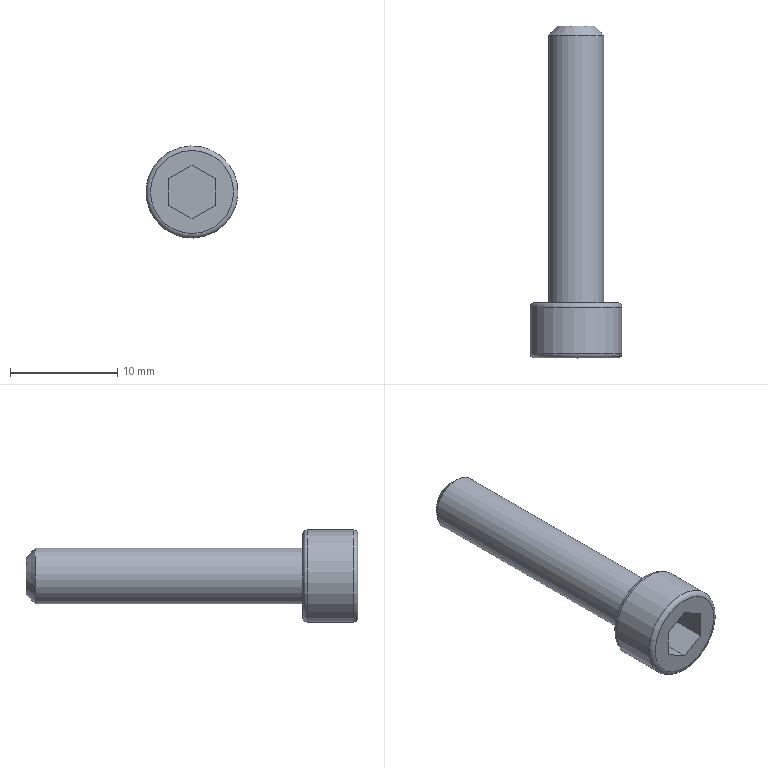Component | NX | M6X30_HEX_SCREW_3 | 1 solid | 15 faces | box 8.6 x 30.96 x 8.6 mm | volume 763 mm3 | plane 10 | cylinder 2 | torus 2 | cone 1 | commonest cylinder face diameters 5.16 x1 8.6 x1
STEP:
#1=CARTESIAN_POINT('',(0.,0.,0.));
#2=DIRECTION('',(0.,0.,1.));
#3=DIRECTION('',(1.,0.,0.));
#4=AXIS2_PLACEMENT_3D('',#1,#2,#3);
#5=CARTESIAN_POINT('',(-9.982,-499.433,-60.987));
#6=VERTEX_POINT('',#5);
#7=CARTESIAN_POINT('',(-11.917,-499.433,-57.635));
#8=DIRECTION('',(0.,-1.,0.));
#9=DIRECTION('',(0.5,0.,-0.866));
#10=AXIS2_PLACEMENT_3D('',#7,#8,#9);
#11=CIRCLE('',#10,3.87);
#12=CARTESIAN_POINT('',(-15.641,-499.433,-59.785));
#13=DIRECTION('',(0.,1.,0.));
#14=DIRECTION('',(0.5,0.,-0.866));
#15=AXIS2_PLACEMENT_3D('',#12,#13,#14);
#16=PLANE('',#15);
#17=CARTESIAN_POINT('',(3.87,-4.3));
#18=CARTESIAN_POINT('',(3.87,-11.003));
#19=CARTESIAN_POINT('',(-1.935,-7.652));
#20=CARTESIAN_POINT('',(-7.74,-4.3));
#21=CARTESIAN_POINT('',(-1.935,-0.9485));
#22=CARTESIAN_POINT('',(3.87,2.403));
#23=CARTESIAN_POINT('',(3.87,-4.3));
#24=(BOUNDED_CURVE()B_SPLINE_CURVE(2,(#17,#18,#19,#20,#21,#22,#23),.UNSPECIFIED.,.T.,.F.)B_SPLINE_CURVE_WITH_KNOTS((1,2,2,2,2,1),(-2.094,0.,2.094,4.189,6.283,8.378),.UNSPECIFIED.)CURVE()GEOMETRIC_REPRESENTATION_ITEM()RATIONAL_B_SPLINE_CURVE((1.,0.5,1.,0.5,1.,0.5,1.))REPRESENTATION_ITEM(''));
#25=(GEOMETRIC_REPRESENTATION_CONTEXT(2)PARAMETRIC_REPRESENTATION_CONTEXT()REPRESENTATION_CONTEXT('',''));
#26=DEFINITIONAL_REPRESENTATION('',(#24),#25);
#27=PCURVE('',#16,#26);
#28=CARTESIAN_POINT('',(-11.917,-499.003,-57.635));
#29=DIRECTION('',(0.,1.,0.));
#30=DIRECTION('',(0.5,0.,-0.866));
#31=AXIS2_PLACEMENT_3D('',#28,#29,#30);
#32=TOROIDAL_SURFACE('',#31,3.87,0.43);
#33=CARTESIAN_POINT('',(6.283,4.712));
#34=DIRECTION('',(-1.,0.));
#35=VECTOR('',#34,1.);
#36=LINE('',#33,#35);
#37=(GEOMETRIC_REPRESENTATION_CONTEXT(2)PARAMETRIC_REPRESENTATION_CONTEXT()REPRESENTATION_CONTEXT('',''));
#38=DEFINITIONAL_REPRESENTATION('',(#36),#37);
#39=PCURVE('',#32,#38);
#40=SURFACE_CURVE('',#11,(#27,#39),.PCURVE_S1.);
#41=EDGE_CURVE('',#6,#6,#40,.T.);
#42=ORIENTED_EDGE('',*,*,#41,.T.);
#43=EDGE_LOOP('',(#42));
#44=FACE_BOUND('',#43,.T.);
#45=CARTESIAN_POINT('',(-11.917,-499.433,-60.118));
#46=VERTEX_POINT('',#45);
#47=CARTESIAN_POINT('',(-9.767,-499.433,-58.877));
#48=VERTEX_POINT('',#47);
#49=CARTESIAN_POINT('',(-12.132,-499.433,-60.242));
#50=DIRECTION('',(0.866,0.,0.5));
#51=VECTOR('',#50,1.);
#52=LINE('',#49,#51);
#53=CARTESIAN_POINT('',(2.15,-2.81));
#54=DIRECTION('',(0.,-1.));
#55=VECTOR('',#54,1.);
#56=LINE('',#53,#55);
#57=(GEOMETRIC_REPRESENTATION_CONTEXT(2)PARAMETRIC_REPRESENTATION_CONTEXT()REPRESENTATION_CONTEXT('',''));
#58=DEFINITIONAL_REPRESENTATION('',(#56),#57);
#59=PCURVE('',#16,#58);
#60=CARTESIAN_POINT('',(-12.132,-495.133,-60.242));
#61=DIRECTION('',(0.5,0.,-0.866));
#62=DIRECTION('',(0.,-1.,0.));
#63=AXIS2_PLACEMENT_3D('',#60,#61,#62);
#64=PLANE('',#63);
#65=CARTESIAN_POINT('',(4.3,0.));
#66=DIRECTION('',(0.,-1.));
#67=VECTOR('',#66,1.);
#68=LINE('',#65,#67);
#69=(GEOMETRIC_REPRESENTATION_CONTEXT(2)PARAMETRIC_REPRESENTATION_CONTEXT()REPRESENTATION_CONTEXT('',''));
#70=DEFINITIONAL_REPRESENTATION('',(#68),#69);
#71=PCURVE('',#64,#70);
#72=SURFACE_CURVE('',#52,(#59,#71),.PCURVE_S1.);
#73=EDGE_CURVE('',#46,#48,#72,.T.);
#74=ORIENTED_EDGE('',*,*,#73,.F.);
#75=CARTESIAN_POINT('',(-14.067,-499.433,-58.877));
#76=VERTEX_POINT('',#75);
#77=CARTESIAN_POINT('',(-14.282,-499.433,-58.752));
#78=DIRECTION('',(0.866,0.,-0.5));
#79=VECTOR('',#78,1.);
#80=LINE('',#77,#79);
#81=CARTESIAN_POINT('',(-0.215,-1.693));
#82=DIRECTION('',(0.866,-0.5));
#83=VECTOR('',#82,1.);
#84=LINE('',#81,#83);
#85=(GEOMETRIC_REPRESENTATION_CONTEXT(2)PARAMETRIC_REPRESENTATION_CONTEXT()REPRESENTATION_CONTEXT('',''));
#86=DEFINITIONAL_REPRESENTATION('',(#84),#85);
#87=PCURVE('',#16,#86);
#88=CARTESIAN_POINT('',(-14.282,-495.133,-58.752));
#89=DIRECTION('',(-0.5,0.,-0.866));
#90=DIRECTION('',(0.866,0.,-0.5));
#91=AXIS2_PLACEMENT_3D('',#88,#89,#90);
#92=PLANE('',#91);
#93=CARTESIAN_POINT('',(0.,4.3));
#94=DIRECTION('',(1.,0.));
#95=VECTOR('',#94,1.);
#96=LINE('',#93,#95);
#97=(GEOMETRIC_REPRESENTATION_CONTEXT(2)PARAMETRIC_REPRESENTATION_CONTEXT()REPRESENTATION_CONTEXT('',''));
#98=DEFINITIONAL_REPRESENTATION('',(#96),#97);
#99=PCURVE('',#92,#98);
#100=SURFACE_CURVE('',#80,(#87,#99),.PCURVE_S1.);
#101=EDGE_CURVE('',#76,#46,#100,.T.);
#102=ORIENTED_EDGE('',*,*,#101,.F.);
#103=CARTESIAN_POINT('',(-14.067,-499.433,-56.394));
#104=VERTEX_POINT('',#103);
#105=CARTESIAN_POINT('',(-14.067,-499.433,-56.146));
#106=DIRECTION('',(-0.,0.,-1.));
#107=VECTOR('',#106,1.);
#108=LINE('',#105,#107);
#109=CARTESIAN_POINT('',(-2.365,-3.183));
#110=DIRECTION('',(0.866,0.5));
#111=VECTOR('',#110,1.);
#112=LINE('',#109,#111);
#113=(GEOMETRIC_REPRESENTATION_CONTEXT(2)PARAMETRIC_REPRESENTATION_CONTEXT()REPRESENTATION_CONTEXT('',''));
#114=DEFINITIONAL_REPRESENTATION('',(#112),#113);
#115=PCURVE('',#16,#114);
#116=CARTESIAN_POINT('',(-14.067,-495.133,-56.146));
#117=DIRECTION('',(-1.,0.,0.));
#118=DIRECTION('',(-0.,0.,-1.));
#119=AXIS2_PLACEMENT_3D('',#116,#117,#118);
#120=PLANE('',#119);
#121=CARTESIAN_POINT('',(0.,4.3));
#122=DIRECTION('',(1.,0.));
#123=VECTOR('',#122,1.);
#124=LINE('',#121,#123);
#125=(GEOMETRIC_REPRESENTATION_CONTEXT(2)PARAMETRIC_REPRESENTATION_CONTEXT()REPRESENTATION_CONTEXT('',''));
#126=DEFINITIONAL_REPRESENTATION('',(#124),#125);
#127=PCURVE('',#120,#126);
#128=SURFACE_CURVE('',#108,(#115,#127),.PCURVE_S1.);
#129=EDGE_CURVE('',#104,#76,#128,.T.);
#130=ORIENTED_EDGE('',*,*,#129,.F.);
#131=CARTESIAN_POINT('',(-11.917,-499.433,-55.153));
#132=VERTEX_POINT('',#131);
#133=CARTESIAN_POINT('',(-11.702,-499.433,-55.029));
#134=DIRECTION('',(-0.866,0.,-0.5));
#135=VECTOR('',#134,1.);
#136=LINE('',#133,#135);
#137=CARTESIAN_POINT('',(-2.15,-5.79));
#138=DIRECTION('',(0.,1.));
#139=VECTOR('',#138,1.);
#140=LINE('',#137,#139);
#141=(GEOMETRIC_REPRESENTATION_CONTEXT(2)PARAMETRIC_REPRESENTATION_CONTEXT()REPRESENTATION_CONTEXT('',''));
#142=DEFINITIONAL_REPRESENTATION('',(#140),#141);
#143=PCURVE('',#16,#142);
#144=CARTESIAN_POINT('',(-11.702,-495.133,-55.029));
#145=DIRECTION('',(-0.5,0.,0.866));
#146=DIRECTION('',(0.,1.,0.));
#147=AXIS2_PLACEMENT_3D('',#144,#145,#146);
#148=PLANE('',#147);
#149=CARTESIAN_POINT('',(-4.3,0.));
#150=DIRECTION('',(0.,1.));
#151=VECTOR('',#150,1.);
#152=LINE('',#149,#151);
#153=(GEOMETRIC_REPRESENTATION_CONTEXT(2)PARAMETRIC_REPRESENTATION_CONTEXT()REPRESENTATION_CONTEXT('',''));
#154=DEFINITIONAL_REPRESENTATION('',(#152),#153);
#155=PCURVE('',#148,#154);
#156=SURFACE_CURVE('',#136,(#143,#155),.PCURVE_S1.);
#157=EDGE_CURVE('',#132,#104,#156,.T.);
#158=ORIENTED_EDGE('',*,*,#157,.F.);
#159=CARTESIAN_POINT('',(-9.767,-499.433,-56.394));
#160=VERTEX_POINT('',#159);
#161=CARTESIAN_POINT('',(-9.552,-499.433,-56.518));
#162=DIRECTION('',(-0.866,0.,0.5));
#163=VECTOR('',#162,1.);
#164=LINE('',#161,#163);
#165=CARTESIAN_POINT('',(0.215,-6.907));
#166=DIRECTION('',(-0.866,0.5));
#167=VECTOR('',#166,1.);
#168=LINE('',#165,#167);
#169=(GEOMETRIC_REPRESENTATION_CONTEXT(2)PARAMETRIC_REPRESENTATION_CONTEXT()REPRESENTATION_CONTEXT('',''));
#170=DEFINITIONAL_REPRESENTATION('',(#168),#169);
#171=PCURVE('',#16,#170);
#172=CARTESIAN_POINT('',(-9.552,-495.133,-56.518));
#173=DIRECTION('',(0.5,0.,0.866));
#174=DIRECTION('',(-0.866,0.,0.5));
#175=AXIS2_PLACEMENT_3D('',#172,#173,#174);
#176=PLANE('',#175);
#177=CARTESIAN_POINT('',(0.,4.3));
#178=DIRECTION('',(1.,0.));
#179=VECTOR('',#178,1.);
#180=LINE('',#177,#179);
#181=(GEOMETRIC_REPRESENTATION_CONTEXT(2)PARAMETRIC_REPRESENTATION_CONTEXT()REPRESENTATION_CONTEXT('',''));
#182=DEFINITIONAL_REPRESENTATION('',(#180),#181);
#183=PCURVE('',#176,#182);
#184=SURFACE_CURVE('',#164,(#171,#183),.PCURVE_S1.);
#185=EDGE_CURVE('',#160,#132,#184,.T.);
#186=ORIENTED_EDGE('',*,*,#185,.F.);
#187=CARTESIAN_POINT('',(-9.767,-499.433,-59.125));
#188=DIRECTION('',(0.,0.,1.));
#189=VECTOR('',#188,1.);
#190=LINE('',#187,#189);
#191=CARTESIAN_POINT('',(2.365,-5.417));
#192=DIRECTION('',(-0.866,-0.5));
#193=VECTOR('',#192,1.);
#194=LINE('',#191,#193);
#195=(GEOMETRIC_REPRESENTATION_CONTEXT(2)PARAMETRIC_REPRESENTATION_CONTEXT()REPRESENTATION_CONTEXT('',''));
#196=DEFINITIONAL_REPRESENTATION('',(#194),#195);
#197=PCURVE('',#16,#196);
#198=CARTESIAN_POINT('',(-9.767,-495.133,-59.125));
#199=DIRECTION('',(1.,0.,-0.));
#200=DIRECTION('',(0.,0.,1.));
#201=AXIS2_PLACEMENT_3D('',#198,#199,#200);
#202=PLANE('',#201);
#203=CARTESIAN_POINT('',(0.,4.3));
#204=DIRECTION('',(1.,0.));
#205=VECTOR('',#204,1.);
#206=LINE('',#203,#205);
#207=(GEOMETRIC_REPRESENTATION_CONTEXT(2)PARAMETRIC_REPRESENTATION_CONTEXT()REPRESENTATION_CONTEXT('',''));
#208=DEFINITIONAL_REPRESENTATION('',(#206),#207);
#209=PCURVE('',#202,#208);
#210=SURFACE_CURVE('',#190,(#197,#209),.PCURVE_S1.);
#211=EDGE_CURVE('',#48,#160,#210,.T.);
#212=ORIENTED_EDGE('',*,*,#211,.F.);
#213=EDGE_LOOP('',(#74,#102,#130,#158,#186,#212));
#214=FACE_BOUND('',#213,.T.);
#215=ADVANCED_FACE('',(#44,#214),#16,.F.);
#216=CARTESIAN_POINT('',(-12.777,-468.473,-56.146));
#217=VERTEX_POINT('',#216);
#218=CARTESIAN_POINT('',(-11.917,-468.473,-57.635));
#219=DIRECTION('',(0.,1.,0.));
#220=DIRECTION('',(-0.5,0.,0.866));
#221=AXIS2_PLACEMENT_3D('',#218,#219,#220);
#222=CIRCLE('',#221,1.72);
#223=CARTESIAN_POINT('',(-11.917,-468.473,-57.635));
#224=DIRECTION('',(0.,-1.,0.));
#225=DIRECTION('',(-0.5,0.,0.866));
#226=AXIS2_PLACEMENT_3D('',#223,#224,#225);
#227=PLANE('',#226);
#228=CARTESIAN_POINT('',(1.72,-0.));
#229=CARTESIAN_POINT('',(1.72,-2.979));
#230=CARTESIAN_POINT('',(-0.86,-1.49));
#231=CARTESIAN_POINT('',(-3.44,0.));
#232=CARTESIAN_POINT('',(-0.86,1.49));
#233=CARTESIAN_POINT('',(1.72,2.979));
#234=CARTESIAN_POINT('',(1.72,-0.));
#235=(BOUNDED_CURVE()B_SPLINE_CURVE(2,(#228,#229,#230,#231,#232,#233,#234),.UNSPECIFIED.,.T.,.F.)B_SPLINE_CURVE_WITH_KNOTS((1,2,2,2,2,1),(-2.094,0.,2.094,4.189,6.283,8.378),.UNSPECIFIED.)CURVE()GEOMETRIC_REPRESENTATION_ITEM()RATIONAL_B_SPLINE_CURVE((1.,0.5,1.,0.5,1.,0.5,1.))REPRESENTATION_ITEM(''));
#236=(GEOMETRIC_REPRESENTATION_CONTEXT(2)PARAMETRIC_REPRESENTATION_CONTEXT()REPRESENTATION_CONTEXT('',''));
#237=DEFINITIONAL_REPRESENTATION('',(#235),#236);
#238=PCURVE('',#227,#237);
#239=CARTESIAN_POINT('',(-11.917,-469.333,-57.635));
#240=DIRECTION('',(0.,-1.,0.));
#241=DIRECTION('',(-0.5,0.,0.866));
#242=AXIS2_PLACEMENT_3D('',#239,#240,#241);
#243=CONICAL_SURFACE('',#242,2.58,0.7854);
#244=CARTESIAN_POINT('',(6.283,-0.86));
#245=DIRECTION('',(-1.,0.));
#246=VECTOR('',#245,1.);
#247=LINE('',#244,#246);
#248=(GEOMETRIC_REPRESENTATION_CONTEXT(2)PARAMETRIC_REPRESENTATION_CONTEXT()REPRESENTATION_CONTEXT('',''));
#249=DEFINITIONAL_REPRESENTATION('',(#247),#248);
#250=PCURVE('',#243,#249);
#251=SURFACE_CURVE('',#222,(#238,#250),.PCURVE_S1.);
#252=EDGE_CURVE('',#217,#217,#251,.T.);
#253=ORIENTED_EDGE('',*,*,#252,.T.);
#254=EDGE_LOOP('',(#253));
#255=FACE_BOUND('',#254,.T.);
#256=ADVANCED_FACE('',(#255),#227,.F.);
#257=CARTESIAN_POINT('',(-13.207,-469.333,-55.401));
#258=VERTEX_POINT('',#257);
#259=CARTESIAN_POINT('',(-11.917,-469.333,-57.635));
#260=DIRECTION('',(0.,-1.,0.));
#261=DIRECTION('',(-0.5,0.,0.866));
#262=AXIS2_PLACEMENT_3D('',#259,#260,#261);
#263=CIRCLE('',#262,2.58);
#264=CARTESIAN_POINT('',(-11.917,-468.473,-57.635));
#265=DIRECTION('',(0.,-1.,0.));
#266=DIRECTION('',(-0.5,0.,0.866));
#267=AXIS2_PLACEMENT_3D('',#264,#265,#266);
#268=CYLINDRICAL_SURFACE('',#267,2.58);
#269=CARTESIAN_POINT('',(0.,0.86));
#270=DIRECTION('',(1.,0.));
#271=VECTOR('',#270,1.);
#272=LINE('',#269,#271);
#273=(GEOMETRIC_REPRESENTATION_CONTEXT(2)PARAMETRIC_REPRESENTATION_CONTEXT()REPRESENTATION_CONTEXT('',''));
#274=DEFINITIONAL_REPRESENTATION('',(#272),#273);
#275=PCURVE('',#268,#274);
#276=CARTESIAN_POINT('',(0.,-0.));
#277=DIRECTION('',(1.,0.));
#278=VECTOR('',#277,1.);
#279=LINE('',#276,#278);
#280=(GEOMETRIC_REPRESENTATION_CONTEXT(2)PARAMETRIC_REPRESENTATION_CONTEXT()REPRESENTATION_CONTEXT('',''));
#281=DEFINITIONAL_REPRESENTATION('',(#279),#280);
#282=PCURVE('',#243,#281);
#283=SURFACE_CURVE('',#263,(#275,#282),.PCURVE_S1.);
#284=EDGE_CURVE('',#258,#258,#283,.T.);
#285=ORIENTED_EDGE('',*,*,#284,.T.);
#286=CARTESIAN_POINT('',(-13.207,-494.273,-55.401));
#287=VERTEX_POINT('',#286);
#288=CARTESIAN_POINT('',(-13.207,-469.333,-55.401));
#289=CARTESIAN_POINT('',(-13.207,-494.273,-55.401));
#290=B_SPLINE_CURVE_WITH_KNOTS('',1,(#288,#289),.UNSPECIFIED.,.F.,.F.,(2,2),(0.86,25.8),.PIECEWISE_BEZIER_KNOTS.);
#291=CARTESIAN_POINT('',(6.283,0.));
#292=DIRECTION('',(0.,1.));
#293=VECTOR('',#292,1.);
#294=LINE('',#291,#293);
#295=(GEOMETRIC_REPRESENTATION_CONTEXT(2)PARAMETRIC_REPRESENTATION_CONTEXT()REPRESENTATION_CONTEXT('',''));
#296=DEFINITIONAL_REPRESENTATION('',(#294),#295);
#297=PCURVE('',#268,#296);
#298=CARTESIAN_POINT('',(0.,0.));
#299=DIRECTION('',(0.,1.));
#300=VECTOR('',#299,1.);
#301=LINE('',#298,#300);
#302=(GEOMETRIC_REPRESENTATION_CONTEXT(2)PARAMETRIC_REPRESENTATION_CONTEXT()REPRESENTATION_CONTEXT('',''));
#303=DEFINITIONAL_REPRESENTATION('',(#301),#302);
#304=PCURVE('',#268,#303);
#305=SEAM_CURVE('',#290,(#297,#304),.PCURVE_S1.);
#306=EDGE_CURVE('',#258,#287,#305,.T.);
#307=ORIENTED_EDGE('',*,*,#306,.T.);
#308=CARTESIAN_POINT('',(-11.917,-494.273,-57.635));
#309=DIRECTION('',(0.,-1.,0.));
#310=DIRECTION('',(-0.5,0.,0.866));
#311=AXIS2_PLACEMENT_3D('',#308,#309,#310);
#312=CIRCLE('',#311,2.58);
#313=CARTESIAN_POINT('',(0.,25.8));
#314=DIRECTION('',(1.,0.));
#315=VECTOR('',#314,1.);
#316=LINE('',#313,#315);
#317=(GEOMETRIC_REPRESENTATION_CONTEXT(2)PARAMETRIC_REPRESENTATION_CONTEXT()REPRESENTATION_CONTEXT('',''));
#318=DEFINITIONAL_REPRESENTATION('',(#316),#317);
#319=PCURVE('',#268,#318);
#320=CARTESIAN_POINT('',(-14.151,-494.273,-58.925));
#321=DIRECTION('',(0.,-1.,0.));
#322=DIRECTION('',(-0.5,0.,0.866));
#323=AXIS2_PLACEMENT_3D('',#320,#321,#322);
#324=PLANE('',#323);
#325=CARTESIAN_POINT('',(-0.,-2.58));
#326=DIRECTION('',(1.,-0.));
#327=AXIS2_PLACEMENT_2D('',#325,#326);
#328=CIRCLE('',#327,2.58);
#329=(GEOMETRIC_REPRESENTATION_CONTEXT(2)PARAMETRIC_REPRESENTATION_CONTEXT()REPRESENTATION_CONTEXT('',''));
#330=DEFINITIONAL_REPRESENTATION('',(#328),#329);
#331=PCURVE('',#324,#330);
#332=SURFACE_CURVE('',#312,(#319,#331),.PCURVE_S1.);
#333=EDGE_CURVE('',#287,#287,#332,.T.);
#334=ORIENTED_EDGE('',*,*,#333,.F.);
#335=ORIENTED_EDGE('',*,*,#306,.F.);
#336=EDGE_LOOP('',(#285,#307,#334,#335));
#337=FACE_BOUND('',#336,.T.);
#338=ADVANCED_FACE('',(#337),#268,.T.);
#339=CARTESIAN_POINT('',(-13.852,-494.273,-54.284));
#340=VERTEX_POINT('',#339);
#341=CARTESIAN_POINT('',(-11.917,-494.273,-57.635));
#342=DIRECTION('',(0.,1.,0.));
#343=DIRECTION('',(-0.5,0.,0.866));
#344=AXIS2_PLACEMENT_3D('',#341,#342,#343);
#345=CIRCLE('',#344,3.87);
#346=CARTESIAN_POINT('',(3.87,-2.58));
#347=CARTESIAN_POINT('',(3.87,-9.283));
#348=CARTESIAN_POINT('',(-1.935,-5.932));
#349=CARTESIAN_POINT('',(-7.74,-2.58));
#350=CARTESIAN_POINT('',(-1.935,0.7715));
#351=CARTESIAN_POINT('',(3.87,4.123));
#352=CARTESIAN_POINT('',(3.87,-2.58));
#353=(BOUNDED_CURVE()B_SPLINE_CURVE(2,(#346,#347,#348,#349,#350,#351,#352),.UNSPECIFIED.,.T.,.F.)B_SPLINE_CURVE_WITH_KNOTS((1,2,2,2,2,1),(-2.094,0.,2.094,4.189,6.283,8.378),.UNSPECIFIED.)CURVE()GEOMETRIC_REPRESENTATION_ITEM()RATIONAL_B_SPLINE_CURVE((1.,0.5,1.,0.5,1.,0.5,1.))REPRESENTATION_ITEM(''));
#354=(GEOMETRIC_REPRESENTATION_CONTEXT(2)PARAMETRIC_REPRESENTATION_CONTEXT()REPRESENTATION_CONTEXT('',''));
#355=DEFINITIONAL_REPRESENTATION('',(#353),#354);
#356=PCURVE('',#324,#355);
#357=CARTESIAN_POINT('',(-11.917,-494.703,-57.635));
#358=DIRECTION('',(0.,-1.,0.));
#359=DIRECTION('',(-0.5,0.,0.866));
#360=AXIS2_PLACEMENT_3D('',#357,#358,#359);
#361=TOROIDAL_SURFACE('',#360,3.87,0.43);
#362=CARTESIAN_POINT('',(6.283,4.712));
#363=DIRECTION('',(-1.,0.));
#364=VECTOR('',#363,1.);
#365=LINE('',#362,#364);
#366=(GEOMETRIC_REPRESENTATION_CONTEXT(2)PARAMETRIC_REPRESENTATION_CONTEXT()REPRESENTATION_CONTEXT('',''));
#367=DEFINITIONAL_REPRESENTATION('',(#365),#366);
#368=PCURVE('',#361,#367);
#369=SURFACE_CURVE('',#345,(#356,#368),.PCURVE_S1.);
#370=EDGE_CURVE('',#340,#340,#369,.T.);
#371=ORIENTED_EDGE('',*,*,#370,.T.);
#372=EDGE_LOOP('',(#371));
#373=FACE_BOUND('',#372,.T.);
#374=ORIENTED_EDGE('',*,*,#333,.T.);
#375=EDGE_LOOP('',(#374));
#376=FACE_BOUND('',#375,.T.);
#377=ADVANCED_FACE('',(#373,#376),#324,.F.);
#378=CARTESIAN_POINT('',(-14.067,-494.703,-53.911));
#379=VERTEX_POINT('',#378);
#380=CARTESIAN_POINT('',(-11.917,-494.703,-57.635));
#381=DIRECTION('',(0.,-1.,0.));
#382=DIRECTION('',(-0.5,0.,0.866));
#383=AXIS2_PLACEMENT_3D('',#380,#381,#382);
#384=CIRCLE('',#383,4.3);
#385=CARTESIAN_POINT('',(-11.917,-468.473,-57.635));
#386=DIRECTION('',(0.,-1.,0.));
#387=DIRECTION('',(-0.5,0.,0.866));
#388=AXIS2_PLACEMENT_3D('',#385,#386,#387);
#389=CYLINDRICAL_SURFACE('',#388,4.3);
#390=CARTESIAN_POINT('',(0.,26.23));
#391=DIRECTION('',(1.,0.));
#392=VECTOR('',#391,1.);
#393=LINE('',#390,#392);
#394=(GEOMETRIC_REPRESENTATION_CONTEXT(2)PARAMETRIC_REPRESENTATION_CONTEXT()REPRESENTATION_CONTEXT('',''));
#395=DEFINITIONAL_REPRESENTATION('',(#393),#394);
#396=PCURVE('',#389,#395);
#397=CARTESIAN_POINT('',(0.,6.283));
#398=DIRECTION('',(1.,0.));
#399=VECTOR('',#398,1.);
#400=LINE('',#397,#399);
#401=(GEOMETRIC_REPRESENTATION_CONTEXT(2)PARAMETRIC_REPRESENTATION_CONTEXT()REPRESENTATION_CONTEXT('',''));
#402=DEFINITIONAL_REPRESENTATION('',(#400),#401);
#403=PCURVE('',#361,#402);
#404=SURFACE_CURVE('',#384,(#396,#403),.PCURVE_S1.);
#405=EDGE_CURVE('',#379,#379,#404,.T.);
#406=ORIENTED_EDGE('',*,*,#405,.T.);
#407=CARTESIAN_POINT('',(-14.067,-499.003,-53.911));
#408=VERTEX_POINT('',#407);
#409=CARTESIAN_POINT('',(-14.067,-494.703,-53.911));
#410=CARTESIAN_POINT('',(-14.067,-499.003,-53.911));
#411=B_SPLINE_CURVE_WITH_KNOTS('',1,(#409,#410),.UNSPECIFIED.,.F.,.F.,(2,2),(26.23,30.53),.PIECEWISE_BEZIER_KNOTS.);
#412=CARTESIAN_POINT('',(6.283,0.));
#413=DIRECTION('',(0.,1.));
#414=VECTOR('',#413,1.);
#415=LINE('',#412,#414);
#416=(GEOMETRIC_REPRESENTATION_CONTEXT(2)PARAMETRIC_REPRESENTATION_CONTEXT()REPRESENTATION_CONTEXT('',''));
#417=DEFINITIONAL_REPRESENTATION('',(#415),#416);
#418=PCURVE('',#389,#417);
#419=CARTESIAN_POINT('',(0.,0.));
#420=DIRECTION('',(0.,1.));
#421=VECTOR('',#420,1.);
#422=LINE('',#419,#421);
#423=(GEOMETRIC_REPRESENTATION_CONTEXT(2)PARAMETRIC_REPRESENTATION_CONTEXT()REPRESENTATION_CONTEXT('',''));
#424=DEFINITIONAL_REPRESENTATION('',(#422),#423);
#425=PCURVE('',#389,#424);
#426=SEAM_CURVE('',#411,(#418,#425),.PCURVE_S1.);
#427=EDGE_CURVE('',#379,#408,#426,.T.);
#428=ORIENTED_EDGE('',*,*,#427,.T.);
#429=CARTESIAN_POINT('',(-9.767,-499.003,-61.359));
#430=VERTEX_POINT('',#429);
#431=CARTESIAN_POINT('',(-11.917,-499.003,-57.635));
#432=DIRECTION('',(0.,1.,0.));
#433=DIRECTION('',(0.5,0.,-0.866));
#434=AXIS2_PLACEMENT_3D('',#431,#432,#433);
#435=CIRCLE('',#434,4.3);
#436=CARTESIAN_POINT('',(9.425,30.53));
#437=DIRECTION('',(-1.,0.));
#438=VECTOR('',#437,1.);
#439=LINE('',#436,#438);
#440=(GEOMETRIC_REPRESENTATION_CONTEXT(2)PARAMETRIC_REPRESENTATION_CONTEXT()REPRESENTATION_CONTEXT('',''));
#441=DEFINITIONAL_REPRESENTATION('',(#439),#440);
#442=PCURVE('',#389,#441);
#443=CARTESIAN_POINT('',(0.,6.283));
#444=DIRECTION('',(1.,0.));
#445=VECTOR('',#444,1.);
#446=LINE('',#443,#445);
#447=(GEOMETRIC_REPRESENTATION_CONTEXT(2)PARAMETRIC_REPRESENTATION_CONTEXT()REPRESENTATION_CONTEXT('',''));
#448=DEFINITIONAL_REPRESENTATION('',(#446),#447);
#449=PCURVE('',#32,#448);
#450=SURFACE_CURVE('',#435,(#442,#449),.PCURVE_S1.);
#451=EDGE_CURVE('',#408,#430,#450,.T.);
#452=ORIENTED_EDGE('',*,*,#451,.T.);
#453=CARTESIAN_POINT('',(-11.917,-499.003,-57.635));
#454=DIRECTION('',(0.,1.,0.));
#455=DIRECTION('',(0.5,0.,-0.866));
#456=AXIS2_PLACEMENT_3D('',#453,#454,#455);
#457=CIRCLE('',#456,4.3);
#458=CARTESIAN_POINT('',(3.142,30.53));
#459=DIRECTION('',(-1.,0.));
#460=VECTOR('',#459,1.);
#461=LINE('',#458,#460);
#462=(GEOMETRIC_REPRESENTATION_CONTEXT(2)PARAMETRIC_REPRESENTATION_CONTEXT()REPRESENTATION_CONTEXT('',''));
#463=DEFINITIONAL_REPRESENTATION('',(#461),#462);
#464=PCURVE('',#389,#463);
#465=CARTESIAN_POINT('',(0.,6.283));
#466=DIRECTION('',(1.,0.));
#467=VECTOR('',#466,1.);
#468=LINE('',#465,#467);
#469=(GEOMETRIC_REPRESENTATION_CONTEXT(2)PARAMETRIC_REPRESENTATION_CONTEXT()REPRESENTATION_CONTEXT('',''));
#470=DEFINITIONAL_REPRESENTATION('',(#468),#469);
#471=PCURVE('',#32,#470);
#472=SURFACE_CURVE('',#457,(#464,#471),.PCURVE_S1.);
#473=EDGE_CURVE('',#430,#408,#472,.T.);
#474=ORIENTED_EDGE('',*,*,#473,.T.);
#475=ORIENTED_EDGE('',*,*,#427,.F.);
#476=EDGE_LOOP('',(#406,#428,#452,#474,#475));
#477=FACE_BOUND('',#476,.T.);
#478=ADVANCED_FACE('',(#477),#389,.T.);
#479=ORIENTED_EDGE('',*,*,#73,.T.);
#480=CARTESIAN_POINT('',(-9.767,-495.133,-58.877));
#481=VERTEX_POINT('',#480);
#482=CARTESIAN_POINT('',(-9.767,-495.133,-58.877));
#483=DIRECTION('',(0.,1.,0.));
#484=VECTOR('',#483,1.);
#485=LINE('',#482,#484);
#486=CARTESIAN_POINT('',(0.,-2.731));
#487=DIRECTION('',(-1.,0.));
#488=VECTOR('',#487,1.);
#489=LINE('',#486,#488);
#490=(GEOMETRIC_REPRESENTATION_CONTEXT(2)PARAMETRIC_REPRESENTATION_CONTEXT()REPRESENTATION_CONTEXT('',''));
#491=DEFINITIONAL_REPRESENTATION('',(#489),#490);
#492=PCURVE('',#64,#491);
#493=CARTESIAN_POINT('',(0.2483,0.));
#494=DIRECTION('',(0.,-1.));
#495=VECTOR('',#494,1.);
#496=LINE('',#493,#495);
#497=(GEOMETRIC_REPRESENTATION_CONTEXT(2)PARAMETRIC_REPRESENTATION_CONTEXT()REPRESENTATION_CONTEXT('',''));
#498=DEFINITIONAL_REPRESENTATION('',(#496),#497);
#499=PCURVE('',#202,#498);
#500=SURFACE_CURVE('',#485,(#492,#499),.PCURVE_S1.);
#501=EDGE_CURVE('',#48,#481,#500,.T.);
#502=ORIENTED_EDGE('',*,*,#501,.T.);
#503=CARTESIAN_POINT('',(-11.917,-495.133,-60.118));
#504=VERTEX_POINT('',#503);
#505=CARTESIAN_POINT('',(-12.132,-495.133,-60.242));
#506=DIRECTION('',(-0.866,0.,-0.5));
#507=VECTOR('',#506,1.);
#508=LINE('',#505,#507);
#509=CARTESIAN_POINT('',(0.,0.));
#510=DIRECTION('',(0.,1.));
#511=VECTOR('',#510,1.);
#512=LINE('',#509,#511);
#513=(GEOMETRIC_REPRESENTATION_CONTEXT(2)PARAMETRIC_REPRESENTATION_CONTEXT()REPRESENTATION_CONTEXT('',''));
#514=DEFINITIONAL_REPRESENTATION('',(#512),#513);
#515=PCURVE('',#64,#514);
#516=CARTESIAN_POINT('',(-11.917,-495.133,-57.635));
#517=DIRECTION('',(0.,-1.,0.));
#518=DIRECTION('',(-0.5,0.,0.866));
#519=AXIS2_PLACEMENT_3D('',#516,#517,#518);
#520=PLANE('',#519);
#521=CARTESIAN_POINT('',(-2.15,1.49));
#522=DIRECTION('',(0.,1.));
#523=VECTOR('',#522,1.);
#524=LINE('',#521,#523);
#525=(GEOMETRIC_REPRESENTATION_CONTEXT(2)PARAMETRIC_REPRESENTATION_CONTEXT()REPRESENTATION_CONTEXT('',''));
#526=DEFINITIONAL_REPRESENTATION('',(#524),#525);
#527=PCURVE('',#520,#526);
#528=SURFACE_CURVE('',#508,(#515,#527),.PCURVE_S1.);
#529=EDGE_CURVE('',#481,#504,#528,.T.);
#530=ORIENTED_EDGE('',*,*,#529,.T.);
#531=CARTESIAN_POINT('',(-11.917,-495.133,-60.118));
#532=DIRECTION('',(0.,1.,0.));
#533=VECTOR('',#532,1.);
#534=LINE('',#531,#533);
#535=CARTESIAN_POINT('',(0.,-0.2483));
#536=DIRECTION('',(-1.,0.));
#537=VECTOR('',#536,1.);
#538=LINE('',#535,#537);
#539=(GEOMETRIC_REPRESENTATION_CONTEXT(2)PARAMETRIC_REPRESENTATION_CONTEXT()REPRESENTATION_CONTEXT('',''));
#540=DEFINITIONAL_REPRESENTATION('',(#538),#539);
#541=PCURVE('',#64,#540);
#542=CARTESIAN_POINT('',(2.731,0.));
#543=DIRECTION('',(0.,-1.));
#544=VECTOR('',#543,1.);
#545=LINE('',#542,#544);
#546=(GEOMETRIC_REPRESENTATION_CONTEXT(2)PARAMETRIC_REPRESENTATION_CONTEXT()REPRESENTATION_CONTEXT('',''));
#547=DEFINITIONAL_REPRESENTATION('',(#545),#546);
#548=PCURVE('',#92,#547);
#549=SURFACE_CURVE('',#534,(#541,#548),.PCURVE_S1.);
#550=EDGE_CURVE('',#46,#504,#549,.T.);
#551=ORIENTED_EDGE('',*,*,#550,.F.);
#552=EDGE_LOOP('',(#479,#502,#530,#551));
#553=FACE_BOUND('',#552,.T.);
#554=ADVANCED_FACE('',(#553),#64,.F.);
#555=ORIENTED_EDGE('',*,*,#211,.T.);
#556=CARTESIAN_POINT('',(-9.767,-495.133,-56.394));
#557=VERTEX_POINT('',#556);
#558=CARTESIAN_POINT('',(-9.767,-495.133,-56.394));
#559=DIRECTION('',(0.,1.,0.));
#560=VECTOR('',#559,1.);
#561=LINE('',#558,#560);
#562=CARTESIAN_POINT('',(2.731,0.));
#563=DIRECTION('',(0.,-1.));
#564=VECTOR('',#563,1.);
#565=LINE('',#562,#564);
#566=(GEOMETRIC_REPRESENTATION_CONTEXT(2)PARAMETRIC_REPRESENTATION_CONTEXT()REPRESENTATION_CONTEXT('',''));
#567=DEFINITIONAL_REPRESENTATION('',(#565),#566);
#568=PCURVE('',#202,#567);
#569=CARTESIAN_POINT('',(0.2483,0.));
#570=DIRECTION('',(0.,-1.));
#571=VECTOR('',#570,1.);
#572=LINE('',#569,#571);
#573=(GEOMETRIC_REPRESENTATION_CONTEXT(2)PARAMETRIC_REPRESENTATION_CONTEXT()REPRESENTATION_CONTEXT('',''));
#574=DEFINITIONAL_REPRESENTATION('',(#572),#573);
#575=PCURVE('',#176,#574);
#576=SURFACE_CURVE('',#561,(#568,#575),.PCURVE_S1.);
#577=EDGE_CURVE('',#160,#557,#576,.T.);
#578=ORIENTED_EDGE('',*,*,#577,.T.);
#579=CARTESIAN_POINT('',(-9.767,-495.133,-59.125));
#580=DIRECTION('',(-0.,0.,-1.));
#581=VECTOR('',#580,1.);
#582=LINE('',#579,#581);
#583=CARTESIAN_POINT('',(0.,0.));
#584=DIRECTION('',(-1.,0.));
#585=VECTOR('',#584,1.);
#586=LINE('',#583,#585);
#587=(GEOMETRIC_REPRESENTATION_CONTEXT(2)PARAMETRIC_REPRESENTATION_CONTEXT()REPRESENTATION_CONTEXT('',''));
#588=DEFINITIONAL_REPRESENTATION('',(#586),#587);
#589=PCURVE('',#202,#588);
#590=CARTESIAN_POINT('',(-2.365,-1.117));
#591=DIRECTION('',(-0.866,0.5));
#592=VECTOR('',#591,1.);
#593=LINE('',#590,#592);
#594=(GEOMETRIC_REPRESENTATION_CONTEXT(2)PARAMETRIC_REPRESENTATION_CONTEXT()REPRESENTATION_CONTEXT('',''));
#595=DEFINITIONAL_REPRESENTATION('',(#593),#594);
#596=PCURVE('',#520,#595);
#597=SURFACE_CURVE('',#582,(#589,#596),.PCURVE_S1.);
#598=EDGE_CURVE('',#557,#481,#597,.T.);
#599=ORIENTED_EDGE('',*,*,#598,.T.);
#600=ORIENTED_EDGE('',*,*,#501,.F.);
#601=EDGE_LOOP('',(#555,#578,#599,#600));
#602=FACE_BOUND('',#601,.T.);
#603=ADVANCED_FACE('',(#602),#202,.F.);
#604=ORIENTED_EDGE('',*,*,#185,.T.);
#605=CARTESIAN_POINT('',(-11.917,-495.133,-55.153));
#606=VERTEX_POINT('',#605);
#607=CARTESIAN_POINT('',(-11.917,-495.133,-55.153));
#608=DIRECTION('',(0.,1.,0.));
#609=VECTOR('',#608,1.);
#610=LINE('',#607,#609);
#611=CARTESIAN_POINT('',(2.731,0.));
#612=DIRECTION('',(0.,-1.));
#613=VECTOR('',#612,1.);
#614=LINE('',#611,#613);
#615=(GEOMETRIC_REPRESENTATION_CONTEXT(2)PARAMETRIC_REPRESENTATION_CONTEXT()REPRESENTATION_CONTEXT('',''));
#616=DEFINITIONAL_REPRESENTATION('',(#614),#615);
#617=PCURVE('',#176,#616);
#618=CARTESIAN_POINT('',(0.,0.2483));
#619=DIRECTION('',(1.,0.));
#620=VECTOR('',#619,1.);
#621=LINE('',#618,#620);
#622=(GEOMETRIC_REPRESENTATION_CONTEXT(2)PARAMETRIC_REPRESENTATION_CONTEXT()REPRESENTATION_CONTEXT('',''));
#623=DEFINITIONAL_REPRESENTATION('',(#621),#622);
#624=PCURVE('',#148,#623);
#625=SURFACE_CURVE('',#610,(#617,#624),.PCURVE_S1.);
#626=EDGE_CURVE('',#132,#606,#625,.T.);
#627=ORIENTED_EDGE('',*,*,#626,.T.);
#628=CARTESIAN_POINT('',(-9.552,-495.133,-56.518));
#629=DIRECTION('',(0.866,0.,-0.5));
#630=VECTOR('',#629,1.);
#631=LINE('',#628,#630);
#632=CARTESIAN_POINT('',(0.,0.));
#633=DIRECTION('',(-1.,0.));
#634=VECTOR('',#633,1.);
#635=LINE('',#632,#634);
#636=(GEOMETRIC_REPRESENTATION_CONTEXT(2)PARAMETRIC_REPRESENTATION_CONTEXT()REPRESENTATION_CONTEXT('',''));
#637=DEFINITIONAL_REPRESENTATION('',(#635),#636);
#638=PCURVE('',#176,#637);
#639=CARTESIAN_POINT('',(-0.215,-2.607));
#640=DIRECTION('',(-0.866,-0.5));
#641=VECTOR('',#640,1.);
#642=LINE('',#639,#641);
#643=(GEOMETRIC_REPRESENTATION_CONTEXT(2)PARAMETRIC_REPRESENTATION_CONTEXT()REPRESENTATION_CONTEXT('',''));
#644=DEFINITIONAL_REPRESENTATION('',(#642),#643);
#645=PCURVE('',#520,#644);
#646=SURFACE_CURVE('',#631,(#638,#645),.PCURVE_S1.);
#647=EDGE_CURVE('',#606,#557,#646,.T.);
#648=ORIENTED_EDGE('',*,*,#647,.T.);
#649=ORIENTED_EDGE('',*,*,#577,.F.);
#650=EDGE_LOOP('',(#604,#627,#648,#649));
#651=FACE_BOUND('',#650,.T.);
#652=ADVANCED_FACE('',(#651),#176,.F.);
#653=ORIENTED_EDGE('',*,*,#157,.T.);
#654=CARTESIAN_POINT('',(-14.067,-495.133,-56.394));
#655=VERTEX_POINT('',#654);
#656=CARTESIAN_POINT('',(-14.067,-495.133,-56.394));
#657=DIRECTION('',(0.,1.,0.));
#658=VECTOR('',#657,1.);
#659=LINE('',#656,#658);
#660=CARTESIAN_POINT('',(0.,2.731));
#661=DIRECTION('',(1.,0.));
#662=VECTOR('',#661,1.);
#663=LINE('',#660,#662);
#664=(GEOMETRIC_REPRESENTATION_CONTEXT(2)PARAMETRIC_REPRESENTATION_CONTEXT()REPRESENTATION_CONTEXT('',''));
#665=DEFINITIONAL_REPRESENTATION('',(#663),#664);
#666=PCURVE('',#148,#665);
#667=CARTESIAN_POINT('',(0.2483,0.));
#668=DIRECTION('',(0.,-1.));
#669=VECTOR('',#668,1.);
#670=LINE('',#667,#669);
#671=(GEOMETRIC_REPRESENTATION_CONTEXT(2)PARAMETRIC_REPRESENTATION_CONTEXT()REPRESENTATION_CONTEXT('',''));
#672=DEFINITIONAL_REPRESENTATION('',(#670),#671);
#673=PCURVE('',#120,#672);
#674=SURFACE_CURVE('',#659,(#666,#673),.PCURVE_S1.);
#675=EDGE_CURVE('',#104,#655,#674,.T.);
#676=ORIENTED_EDGE('',*,*,#675,.T.);
#677=CARTESIAN_POINT('',(-11.702,-495.133,-55.029));
#678=DIRECTION('',(0.866,0.,0.5));
#679=VECTOR('',#678,1.);
#680=LINE('',#677,#679);
#681=CARTESIAN_POINT('',(0.,0.));
#682=DIRECTION('',(0.,-1.));
#683=VECTOR('',#682,1.);
#684=LINE('',#681,#683);
#685=(GEOMETRIC_REPRESENTATION_CONTEXT(2)PARAMETRIC_REPRESENTATION_CONTEXT()REPRESENTATION_CONTEXT('',''));
#686=DEFINITIONAL_REPRESENTATION('',(#684),#685);
#687=PCURVE('',#148,#686);
#688=CARTESIAN_POINT('',(2.15,-1.49));
#689=DIRECTION('',(0.,-1.));
#690=VECTOR('',#689,1.);
#691=LINE('',#688,#690);
#692=(GEOMETRIC_REPRESENTATION_CONTEXT(2)PARAMETRIC_REPRESENTATION_CONTEXT()REPRESENTATION_CONTEXT('',''));
#693=DEFINITIONAL_REPRESENTATION('',(#691),#692);
#694=PCURVE('',#520,#693);
#695=SURFACE_CURVE('',#680,(#687,#694),.PCURVE_S1.);
#696=EDGE_CURVE('',#655,#606,#695,.T.);
#697=ORIENTED_EDGE('',*,*,#696,.T.);
#698=ORIENTED_EDGE('',*,*,#626,.F.);
#699=EDGE_LOOP('',(#653,#676,#697,#698));
#700=FACE_BOUND('',#699,.T.);
#701=ADVANCED_FACE('',(#700),#148,.F.);
#702=ORIENTED_EDGE('',*,*,#129,.T.);
#703=CARTESIAN_POINT('',(-14.067,-495.133,-58.877));
#704=VERTEX_POINT('',#703);
#705=CARTESIAN_POINT('',(-14.067,-495.133,-58.877));
#706=DIRECTION('',(0.,1.,0.));
#707=VECTOR('',#706,1.);
#708=LINE('',#705,#707);
#709=CARTESIAN_POINT('',(2.731,0.));
#710=DIRECTION('',(0.,-1.));
#711=VECTOR('',#710,1.);
#712=LINE('',#709,#711);
#713=(GEOMETRIC_REPRESENTATION_CONTEXT(2)PARAMETRIC_REPRESENTATION_CONTEXT()REPRESENTATION_CONTEXT('',''));
#714=DEFINITIONAL_REPRESENTATION('',(#712),#713);
#715=PCURVE('',#120,#714);
#716=CARTESIAN_POINT('',(0.2483,0.));
#717=DIRECTION('',(0.,-1.));
#718=VECTOR('',#717,1.);
#719=LINE('',#716,#718);
#720=(GEOMETRIC_REPRESENTATION_CONTEXT(2)PARAMETRIC_REPRESENTATION_CONTEXT()REPRESENTATION_CONTEXT('',''));
#721=DEFINITIONAL_REPRESENTATION('',(#719),#720);
#722=PCURVE('',#92,#721);
#723=SURFACE_CURVE('',#708,(#715,#722),.PCURVE_S1.);
#724=EDGE_CURVE('',#76,#704,#723,.T.);
#725=ORIENTED_EDGE('',*,*,#724,.T.);
#726=CARTESIAN_POINT('',(-14.067,-495.133,-56.146));
#727=DIRECTION('',(0.,0.,1.));
#728=VECTOR('',#727,1.);
#729=LINE('',#726,#728);
#730=CARTESIAN_POINT('',(0.,0.));
#731=DIRECTION('',(-1.,0.));
#732=VECTOR('',#731,1.);
#733=LINE('',#730,#732);
#734=(GEOMETRIC_REPRESENTATION_CONTEXT(2)PARAMETRIC_REPRESENTATION_CONTEXT()REPRESENTATION_CONTEXT('',''));
#735=DEFINITIONAL_REPRESENTATION('',(#733),#734);
#736=PCURVE('',#120,#735);
#737=CARTESIAN_POINT('',(2.365,1.117));
#738=DIRECTION('',(0.866,-0.5));
#739=VECTOR('',#738,1.);
#740=LINE('',#737,#739);
#741=(GEOMETRIC_REPRESENTATION_CONTEXT(2)PARAMETRIC_REPRESENTATION_CONTEXT()REPRESENTATION_CONTEXT('',''));
#742=DEFINITIONAL_REPRESENTATION('',(#740),#741);
#743=PCURVE('',#520,#742);
#744=SURFACE_CURVE('',#729,(#736,#743),.PCURVE_S1.);
#745=EDGE_CURVE('',#704,#655,#744,.T.);
#746=ORIENTED_EDGE('',*,*,#745,.T.);
#747=ORIENTED_EDGE('',*,*,#675,.F.);
#748=EDGE_LOOP('',(#702,#725,#746,#747));
#749=FACE_BOUND('',#748,.T.);
#750=ADVANCED_FACE('',(#749),#120,.F.);
#751=ORIENTED_EDGE('',*,*,#101,.T.);
#752=ORIENTED_EDGE('',*,*,#550,.T.);
#753=CARTESIAN_POINT('',(-14.282,-495.133,-58.752));
#754=DIRECTION('',(-0.866,0.,0.5));
#755=VECTOR('',#754,1.);
#756=LINE('',#753,#755);
#757=CARTESIAN_POINT('',(0.,0.));
#758=DIRECTION('',(-1.,0.));
#759=VECTOR('',#758,1.);
#760=LINE('',#757,#759);
#761=(GEOMETRIC_REPRESENTATION_CONTEXT(2)PARAMETRIC_REPRESENTATION_CONTEXT()REPRESENTATION_CONTEXT('',''));
#762=DEFINITIONAL_REPRESENTATION('',(#760),#761);
#763=PCURVE('',#92,#762);
#764=CARTESIAN_POINT('',(0.215,2.607));
#765=DIRECTION('',(0.866,0.5));
#766=VECTOR('',#765,1.);
#767=LINE('',#764,#766);
#768=(GEOMETRIC_REPRESENTATION_CONTEXT(2)PARAMETRIC_REPRESENTATION_CONTEXT()REPRESENTATION_CONTEXT('',''));
#769=DEFINITIONAL_REPRESENTATION('',(#767),#768);
#770=PCURVE('',#520,#769);
#771=SURFACE_CURVE('',#756,(#763,#770),.PCURVE_S1.);
#772=EDGE_CURVE('',#504,#704,#771,.T.);
#773=ORIENTED_EDGE('',*,*,#772,.T.);
#774=ORIENTED_EDGE('',*,*,#724,.F.);
#775=EDGE_LOOP('',(#751,#752,#773,#774));
#776=FACE_BOUND('',#775,.T.);
#777=ADVANCED_FACE('',(#776),#92,.F.);
#778=ORIENTED_EDGE('',*,*,#529,.F.);
#779=ORIENTED_EDGE('',*,*,#598,.F.);
#780=ORIENTED_EDGE('',*,*,#647,.F.);
#781=ORIENTED_EDGE('',*,*,#696,.F.);
#782=ORIENTED_EDGE('',*,*,#745,.F.);
#783=ORIENTED_EDGE('',*,*,#772,.F.);
#784=EDGE_LOOP('',(#778,#779,#780,#781,#782,#783));
#785=FACE_BOUND('',#784,.T.);
#786=ADVANCED_FACE('',(#785),#520,.T.);
#787=ORIENTED_EDGE('',*,*,#370,.F.);
#788=CARTESIAN_POINT('',(-13.852,-494.273,-54.284));
#789=CARTESIAN_POINT('',(-13.909,-494.273,-54.184));
#790=CARTESIAN_POINT('',(-13.965,-494.31,-54.087));
#791=CARTESIAN_POINT('',(-14.014,-494.38,-54.004));
#792=CARTESIAN_POINT('',(-14.049,-494.476,-53.943));
#793=CARTESIAN_POINT('',(-14.067,-494.588,-53.911));
#794=CARTESIAN_POINT('',(-14.067,-494.703,-53.911));
#795=(BOUNDED_CURVE()B_SPLINE_CURVE(6,(#788,#789,#790,#791,#792,#793,#794),.UNSPECIFIED.,.F.,.F.)B_SPLINE_CURVE_WITH_KNOTS((7,7),(4.712,6.283),.PIECEWISE_BEZIER_KNOTS.)CURVE()GEOMETRIC_REPRESENTATION_ITEM()RATIONAL_B_SPLINE_CURVE((1.031,1.01,0.9979,0.994,0.9979,1.01,1.031))REPRESENTATION_ITEM(''));
#796=CARTESIAN_POINT('',(6.283,0.));
#797=DIRECTION('',(0.,1.));
#798=VECTOR('',#797,1.);
#799=LINE('',#796,#798);
#800=(GEOMETRIC_REPRESENTATION_CONTEXT(2)PARAMETRIC_REPRESENTATION_CONTEXT()REPRESENTATION_CONTEXT('',''));
#801=DEFINITIONAL_REPRESENTATION('',(#799),#800);
#802=PCURVE('',#361,#801);
#803=CARTESIAN_POINT('',(0.,0.));
#804=DIRECTION('',(0.,1.));
#805=VECTOR('',#804,1.);
#806=LINE('',#803,#805);
#807=(GEOMETRIC_REPRESENTATION_CONTEXT(2)PARAMETRIC_REPRESENTATION_CONTEXT()REPRESENTATION_CONTEXT('',''));
#808=DEFINITIONAL_REPRESENTATION('',(#806),#807);
#809=PCURVE('',#361,#808);
#810=SEAM_CURVE('',#795,(#802,#809),.PCURVE_S1.);
#811=EDGE_CURVE('',#340,#379,#810,.T.);
#812=ORIENTED_EDGE('',*,*,#811,.T.);
#813=ORIENTED_EDGE('',*,*,#405,.F.);
#814=ORIENTED_EDGE('',*,*,#811,.F.);
#815=EDGE_LOOP('',(#787,#812,#813,#814));
#816=FACE_BOUND('',#815,.T.);
#817=ADVANCED_FACE('',(#816),#361,.T.);
#818=ORIENTED_EDGE('',*,*,#473,.F.);
#819=CARTESIAN_POINT('',(-9.982,-499.433,-60.987));
#820=CARTESIAN_POINT('',(-9.924,-499.433,-61.086));
#821=CARTESIAN_POINT('',(-9.868,-499.396,-61.183));
#822=CARTESIAN_POINT('',(-9.82,-499.326,-61.267));
#823=CARTESIAN_POINT('',(-9.785,-499.23,-61.328));
#824=CARTESIAN_POINT('',(-9.767,-499.118,-61.359));
#825=CARTESIAN_POINT('',(-9.767,-499.003,-61.359));
#826=(BOUNDED_CURVE()B_SPLINE_CURVE(6,(#819,#820,#821,#822,#823,#824,#825),.UNSPECIFIED.,.F.,.F.)B_SPLINE_CURVE_WITH_KNOTS((7,7),(-1.571,0.),.PIECEWISE_BEZIER_KNOTS.)CURVE()GEOMETRIC_REPRESENTATION_ITEM()RATIONAL_B_SPLINE_CURVE((1.031,1.01,0.9979,0.994,0.9979,1.01,1.031))REPRESENTATION_ITEM(''));
#827=CARTESIAN_POINT('',(0.,6.283));
#828=DIRECTION('',(0.,1.));
#829=VECTOR('',#828,1.);
#830=LINE('',#827,#829);
#831=(GEOMETRIC_REPRESENTATION_CONTEXT(2)PARAMETRIC_REPRESENTATION_CONTEXT()REPRESENTATION_CONTEXT('',''));
#832=DEFINITIONAL_REPRESENTATION('',(#830),#831);
#833=PCURVE('',#32,#832);
#834=CARTESIAN_POINT('',(6.283,6.283));
#835=DIRECTION('',(0.,1.));
#836=VECTOR('',#835,1.);
#837=LINE('',#834,#836);
#838=(GEOMETRIC_REPRESENTATION_CONTEXT(2)PARAMETRIC_REPRESENTATION_CONTEXT()REPRESENTATION_CONTEXT('',''));
#839=DEFINITIONAL_REPRESENTATION('',(#837),#838);
#840=PCURVE('',#32,#839);
#841=SEAM_CURVE('',#826,(#833,#840),.PCURVE_S1.);
#842=EDGE_CURVE('',#6,#430,#841,.T.);
#843=ORIENTED_EDGE('',*,*,#842,.F.);
#844=ORIENTED_EDGE('',*,*,#41,.F.);
#845=ORIENTED_EDGE('',*,*,#842,.T.);
#846=ORIENTED_EDGE('',*,*,#451,.F.);
#847=EDGE_LOOP('',(#818,#843,#844,#845,#846));
#848=FACE_BOUND('',#847,.T.);
#849=ADVANCED_FACE('',(#848),#32,.T.);
#850=ORIENTED_EDGE('',*,*,#252,.F.);
#851=CARTESIAN_POINT('',(-12.777,-468.473,-56.146));
#852=CARTESIAN_POINT('',(-13.207,-469.333,-55.401));
#853=B_SPLINE_CURVE_WITH_KNOTS('',1,(#851,#852),.UNSPECIFIED.,.F.,.F.,(2,2),(-1.216,-0.),.PIECEWISE_BEZIER_KNOTS.);
#854=CARTESIAN_POINT('',(6.283,0.));
#855=DIRECTION('',(0.,1.));
#856=VECTOR('',#855,1.);
#857=LINE('',#854,#856);
#858=(GEOMETRIC_REPRESENTATION_CONTEXT(2)PARAMETRIC_REPRESENTATION_CONTEXT()REPRESENTATION_CONTEXT('',''));
#859=DEFINITIONAL_REPRESENTATION('',(#857),#858);
#860=PCURVE('',#243,#859);
#861=CARTESIAN_POINT('',(0.,0.));
#862=DIRECTION('',(0.,1.));
#863=VECTOR('',#862,1.);
#864=LINE('',#861,#863);
#865=(GEOMETRIC_REPRESENTATION_CONTEXT(2)PARAMETRIC_REPRESENTATION_CONTEXT()REPRESENTATION_CONTEXT('',''));
#866=DEFINITIONAL_REPRESENTATION('',(#864),#865);
#867=PCURVE('',#243,#866);
#868=SEAM_CURVE('',#853,(#860,#867),.PCURVE_S1.);
#869=EDGE_CURVE('',#217,#258,#868,.T.);
#870=ORIENTED_EDGE('',*,*,#869,.T.);
#871=ORIENTED_EDGE('',*,*,#284,.F.);
#872=ORIENTED_EDGE('',*,*,#869,.F.);
#873=EDGE_LOOP('',(#850,#870,#871,#872));
#874=FACE_BOUND('',#873,.T.);
#875=ADVANCED_FACE('',(#874),#243,.T.);
#876=CLOSED_SHELL('',(#215,#256,#338,#377,#478,#554,#603,#652,#701,#750,#777,#786,#817,#849,#875));
#877=MANIFOLD_SOLID_BREP('',#876);
#878=(LENGTH_UNIT()NAMED_UNIT(*)SI_UNIT(.MILLI.,.METRE.));
#879=UNCERTAINTY_MEASURE_WITH_UNIT(LENGTH_MEASURE(0.000002),#878,'','');
#880=(NAMED_UNIT(*)PLANE_ANGLE_UNIT()SI_UNIT($,.RADIAN.));
#881=(NAMED_UNIT(*)SI_UNIT($,.STERADIAN.)SOLID_ANGLE_UNIT());
#882=(GEOMETRIC_REPRESENTATION_CONTEXT(3)GLOBAL_UNCERTAINTY_ASSIGNED_CONTEXT((#879))GLOBAL_UNIT_ASSIGNED_CONTEXT((#878,#880,#881))REPRESENTATION_CONTEXT('',''));
#883=ADVANCED_BREP_SHAPE_REPRESENTATION('',(#4,#877),#882);